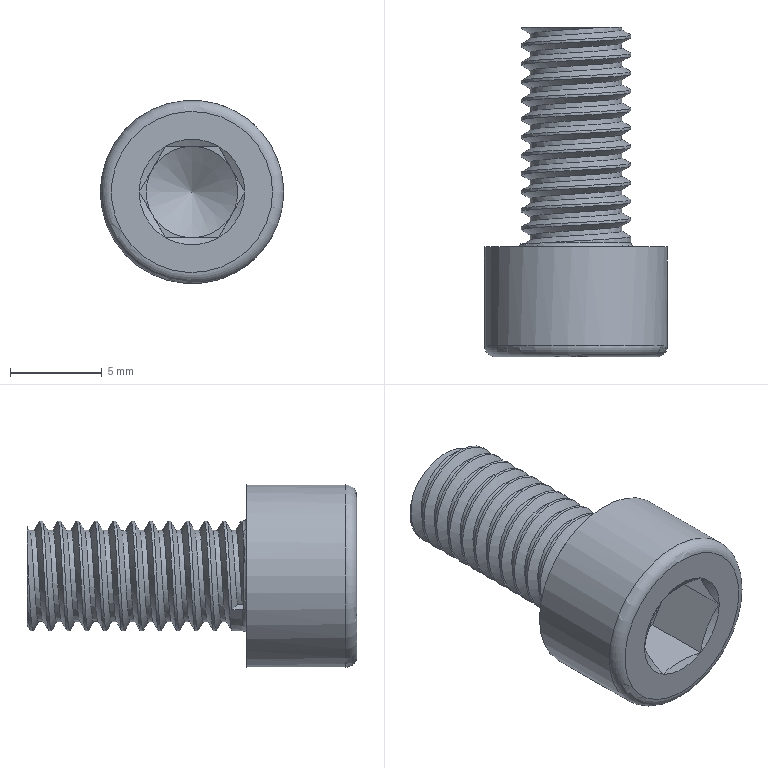Component | NX | M6X12_INT | 1 solid | 31 faces | volume 669 mm3 | plane 16 | cone 7 | cylinder 3 | spline 3 | torus 2 | commonest cylinder face diameters 6 x1 10 x1 5 x1